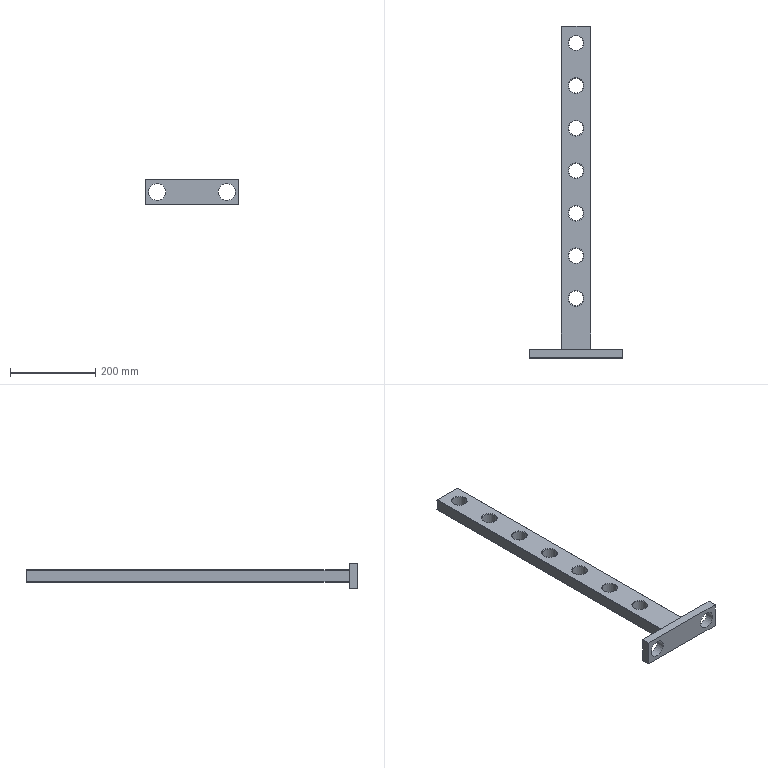Component | NX | A_PART_3 | 1 solid | 54 faces | volume 1538116 mm3 | cylinder 21 | torus 14 | plane 11 | sphere 8 | commonest cylinder face diameters 2 x12 35 x7 40 x2